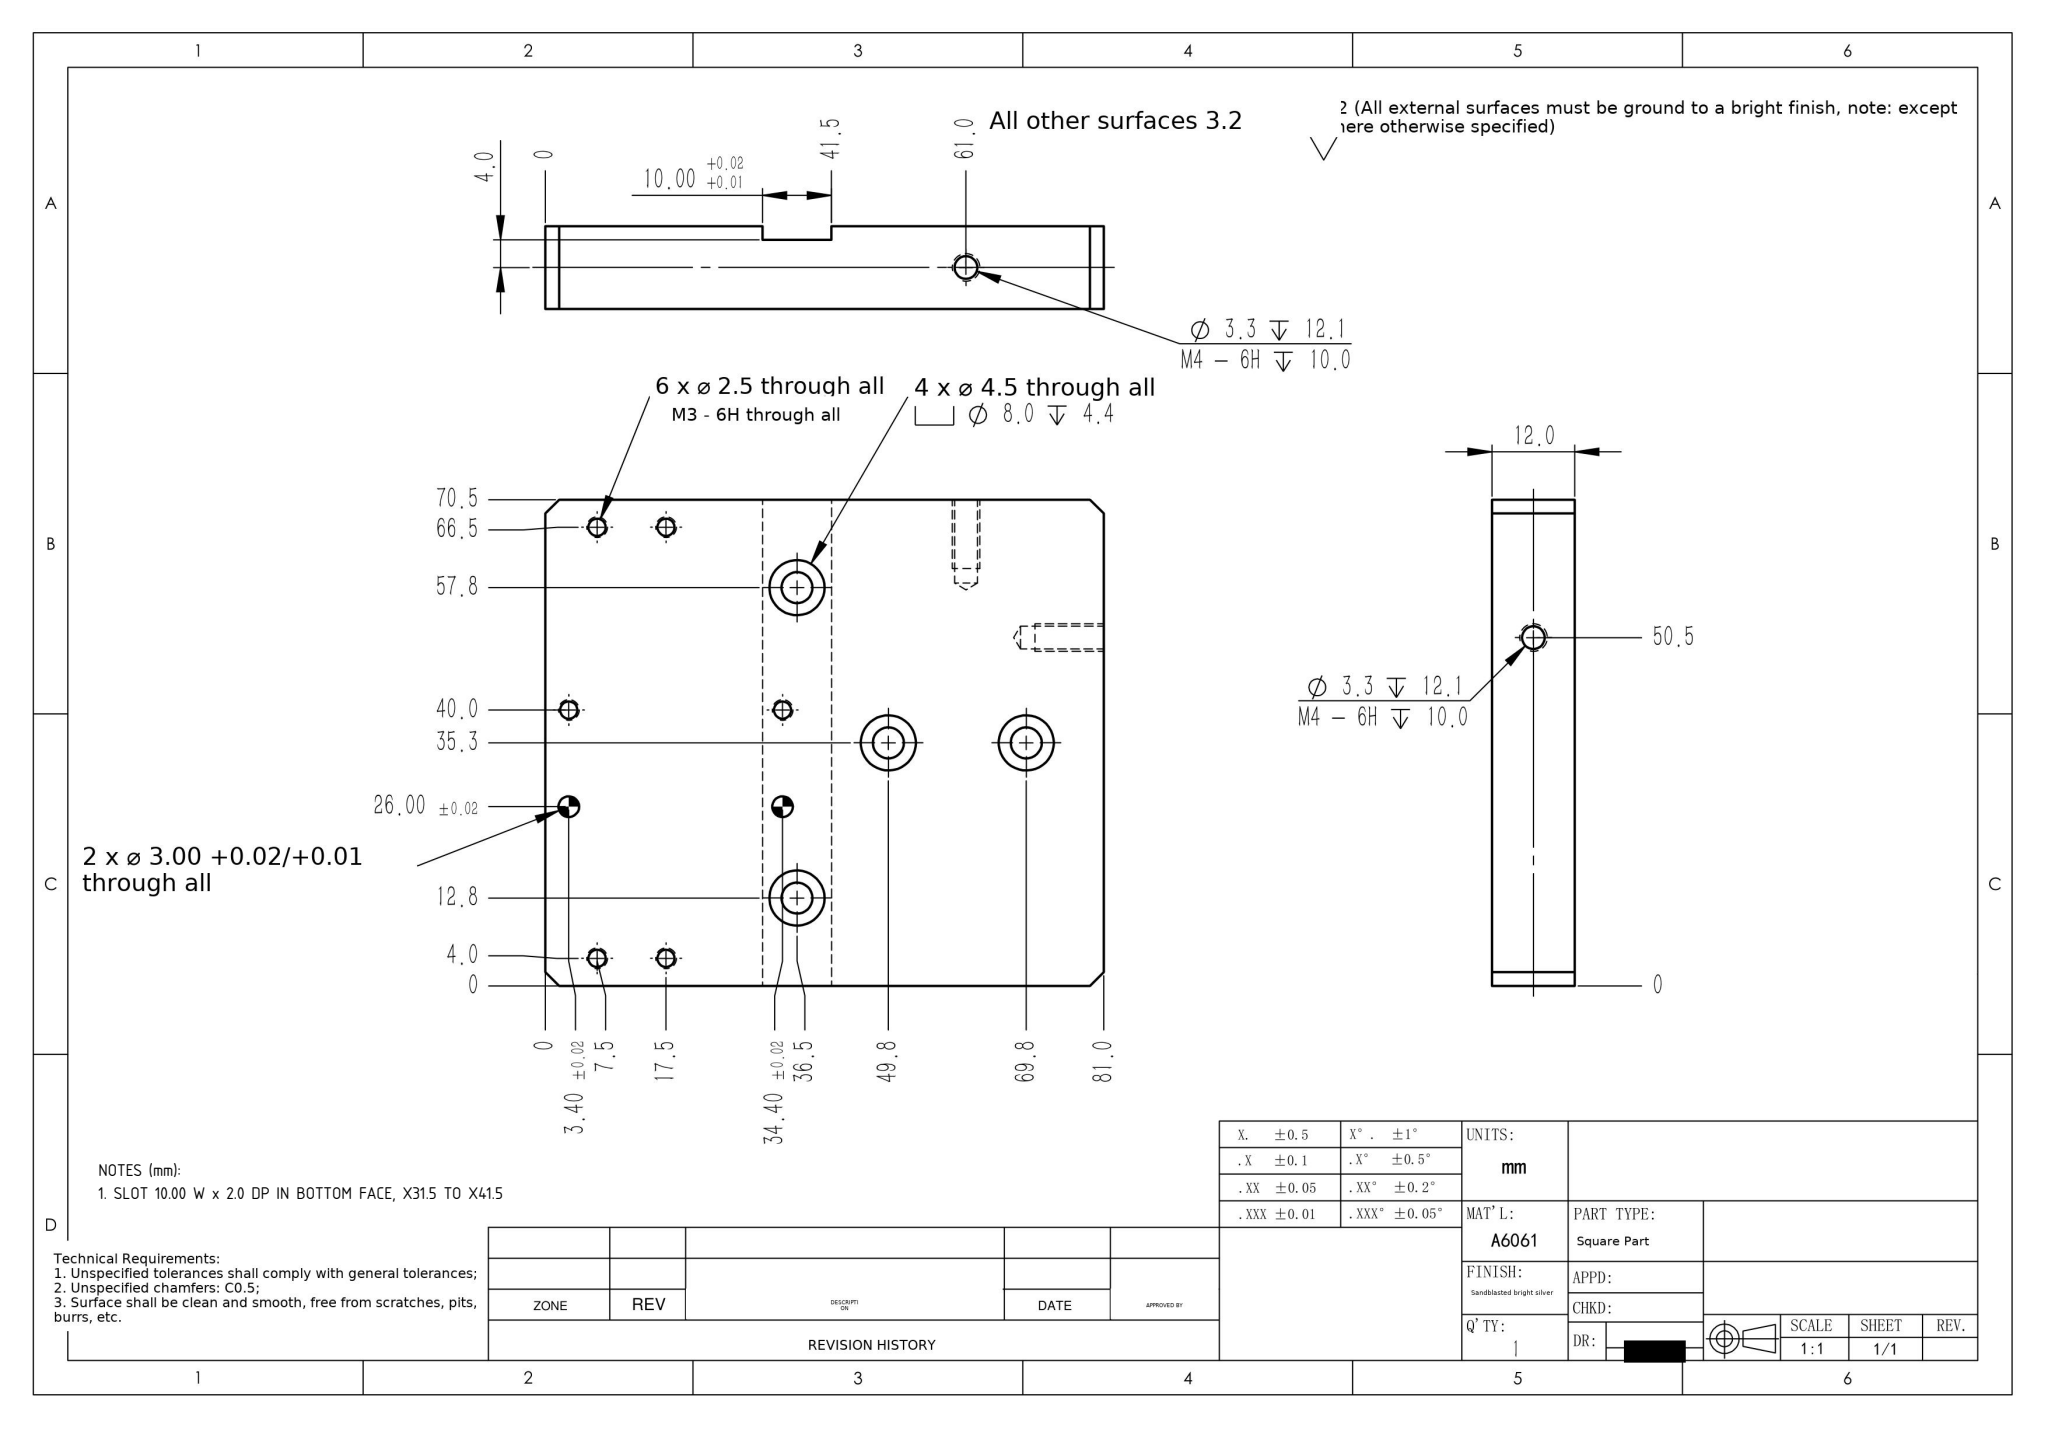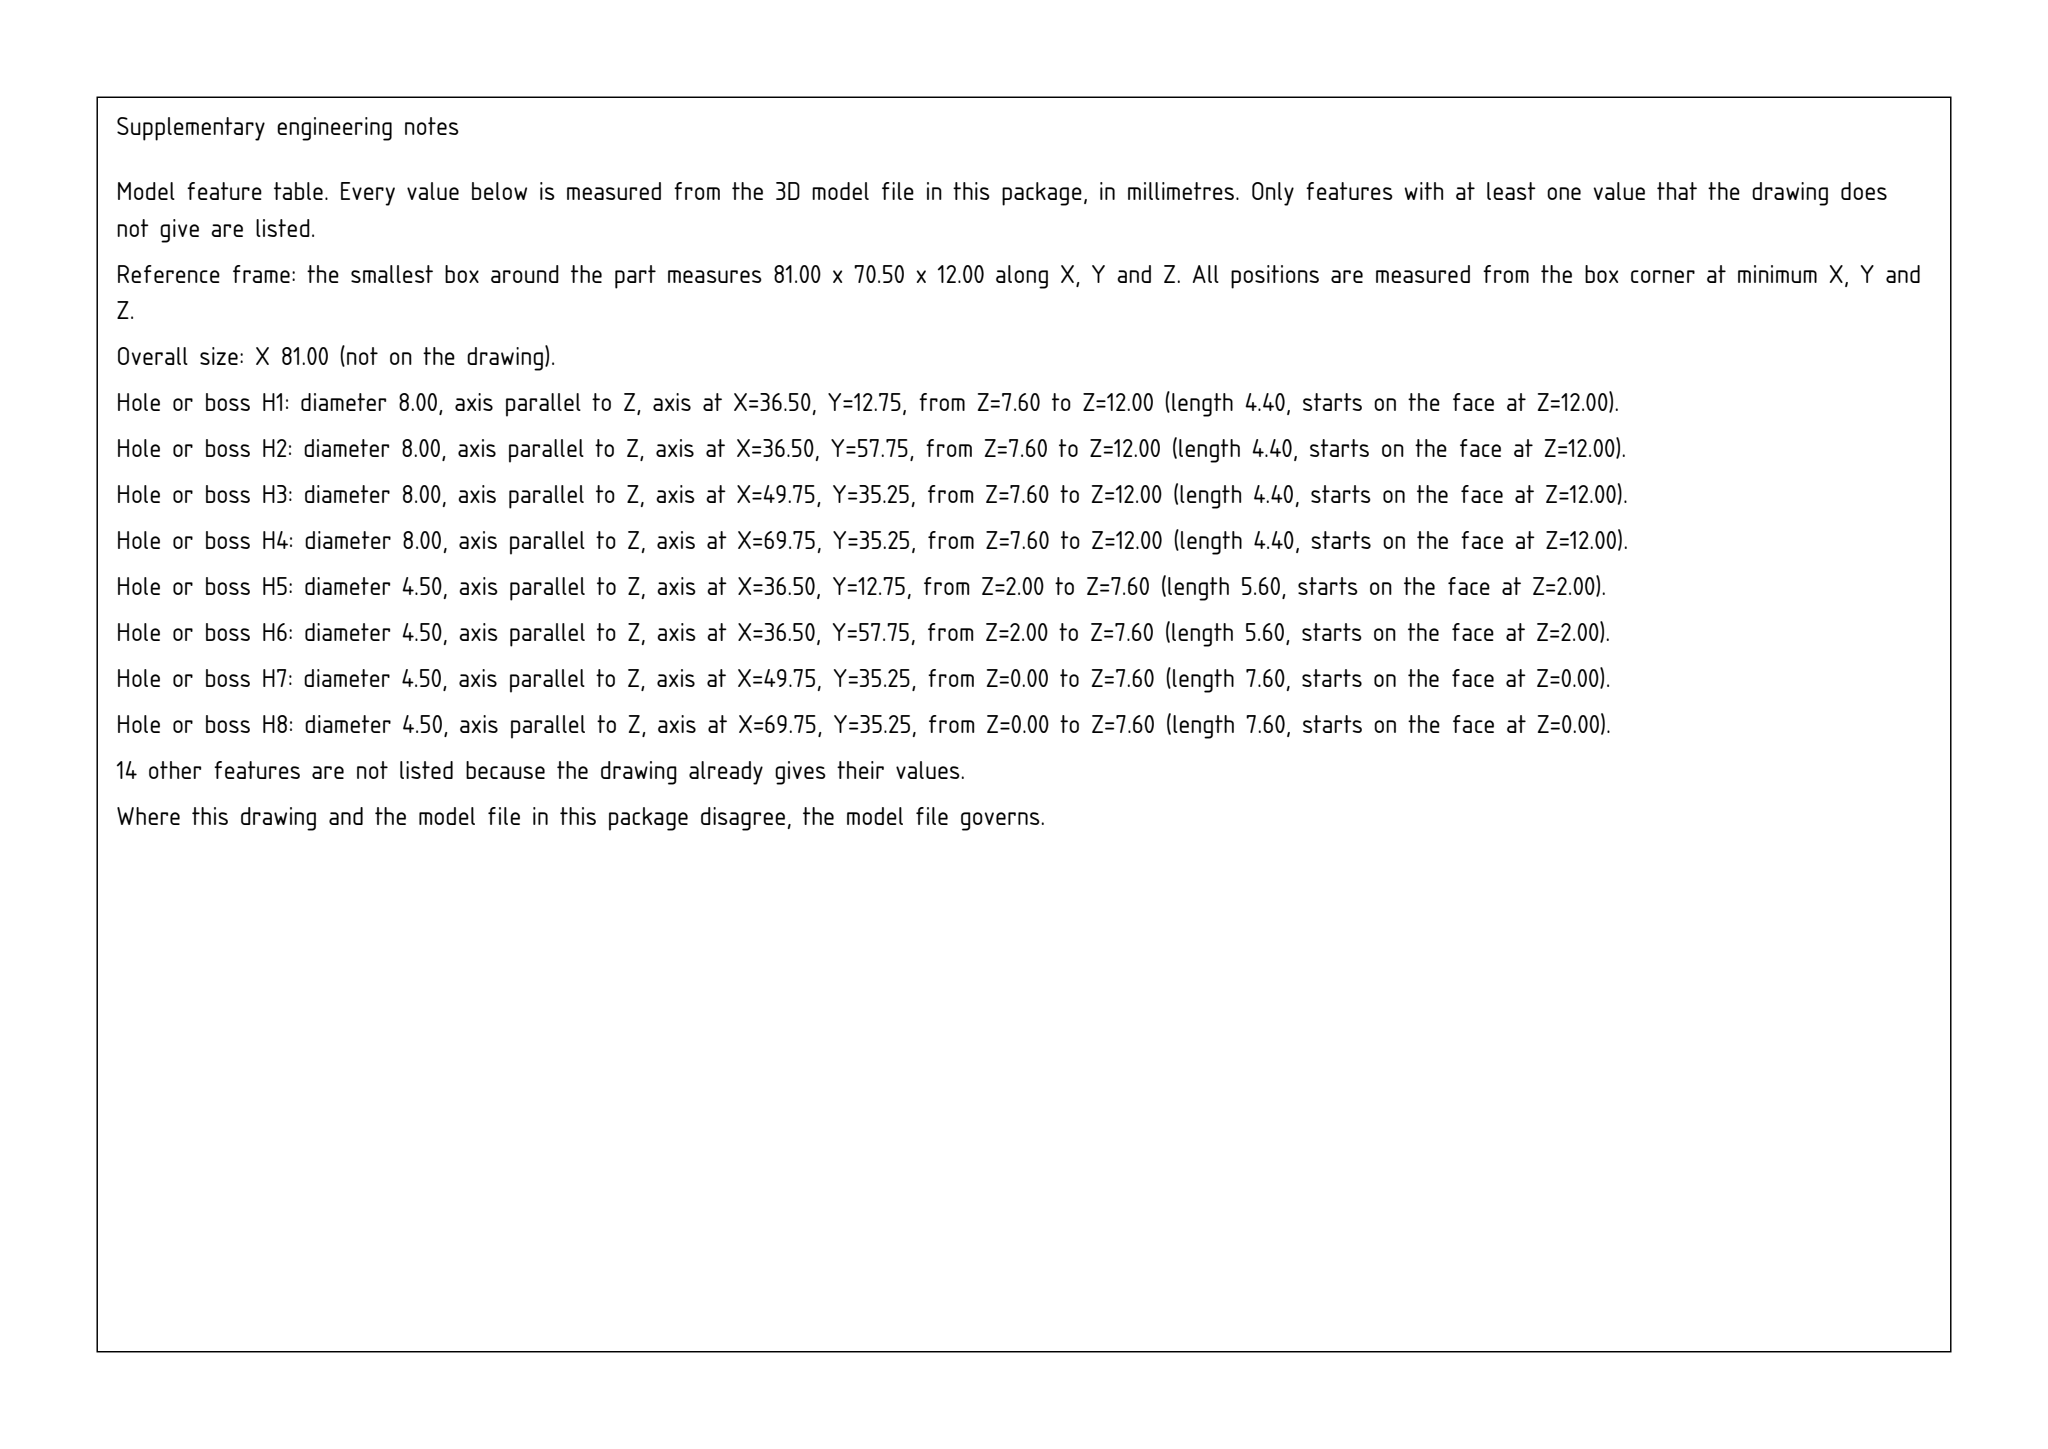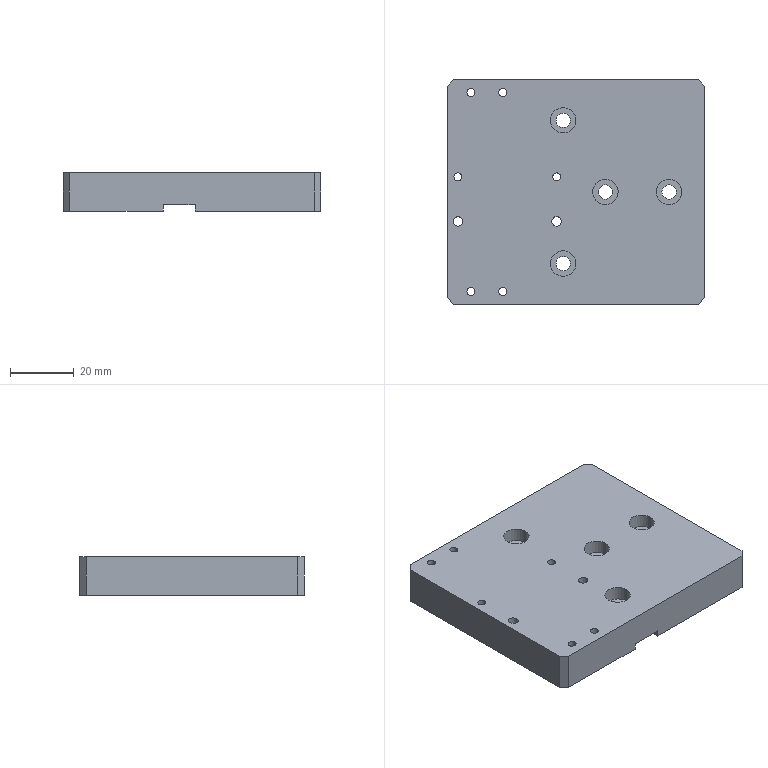Part | SolidWorks | mm | 1 solid | 58 faces | box 81 x 70.5 x 12 mm | volume 65004 mm3 | cylinder 36 | plane 18 | cone 4 | commonest cylinder face diameters 2.5 x12 8 x8 4.5 x8 3.3 x4 3 x4
Drawing notes:
SLOT 10.00 W x 2.0 DP IN BOTTOM FACE, X31.5 TO X41.5 | from the solid: x-planes 31.5 & 41.5 (10.00 wide); z-plane at 2.0 vs 12.0 thk = 2.0 DP cut from z=0 face; Ø2.5 at x=34.4 only 10.0 long and Ø4.5 at x=36.5 5.6 long under 4.4 CBORE (4.4+5.6=10.0)
build123d program:
from build123d import *

# Parameters (mm, degrees)
SKETCH1_W                                       = 81
SKETCH1_H                                       = 70.5
BOSS_EXTRUDE1_DEPTH                             = 12
M4_HEX_SOCKET_HEAD_CAP_SCREW_CBORE1_D           = 4.5
M4_HEX_SOCKET_HEAD_CAP_SCREW_CBORE1_CBORE_D     = 8
M4_HEX_SOCKET_HEAD_CAP_SCREW_CBORE1_CBORE_DEPTH = 4.4
M3_TAPPED_HOLE1_D                               = 2.5
SIZE_MM_DOWEL_PIN_HOLE1_D                       = 3
M4_TAPPED_HOLE1_D                               = 3.3
M4_TAPPED_HOLE1_DEPTH                           = 12.1
M4_TAPPED_HOLE1_TIP                             = 0.9914
M4_TAPPED_HOLE2_D                               = 3.3
M4_TAPPED_HOLE2_DEPTH                           = 12.1
M4_TAPPED_HOLE2_TIP                             = 0.9914
CHAMFER1_SIZE                                   = 2
SKETCH12_W                                      = 10
SKETCH12_H                                      = 70.5
CUT_EXTRUDE1_DEPTH                              = 2


with BuildPart() as part:
    # Sketch1 → Boss-Extrude1 (new body)
    with BuildSketch(Plane.XY):
        Rectangle(SKETCH1_W, SKETCH1_H)
    extrude(amount=BOSS_EXTRUDE1_DEPTH)

    # M4 Hex Socket Head Cap Screw CBORE1 (through all)
    with Locations(Plane.XY.offset(12)):
        with Locations((29.25, 0), (9.25, 0), (-4, 22.5), (-4, -22.5)):
            CounterBoreHole(M4_HEX_SOCKET_HEAD_CAP_SCREW_CBORE1_D / 2, M4_HEX_SOCKET_HEAD_CAP_SCREW_CBORE1_CBORE_D / 2, M4_HEX_SOCKET_HEAD_CAP_SCREW_CBORE1_CBORE_DEPTH)

    # M3 Tapped Hole1 (through all)
    with Locations(Plane.XY.offset(12)):
        with Locations((-33, 31.25), (-23, 31.25), (-23, -31.25), (-33, -31.25), (-37.1, 4.75), (-6.1, 4.75), (-68.1, 4.75)):
            Hole(M3_TAPPED_HOLE1_D / 2)

    # Size mm Dowel Pin Hole1 (through all)
    with Locations(Plane.XY.offset(12)):
        with Locations((-37.1, -9.25), (-6.1, -9.25)):
            Hole(SIZE_MM_DOWEL_PIN_HOLE1_D / 2)

    # M4 Tapped Hole1
    with Locations(Plane(origin=(0, 35.25, 0), x_dir=(1, 0, 0), z_dir=(0, 1, 0))):
        with Locations((20.5, -6)):
            Hole(M4_TAPPED_HOLE1_D / 2, depth=M4_TAPPED_HOLE1_DEPTH)
            with Locations((0, 0, -(M4_TAPPED_HOLE1_DEPTH + M4_TAPPED_HOLE1_TIP / 2))):  # 118° drill point
                Cone(0, M4_TAPPED_HOLE1_D / 2, M4_TAPPED_HOLE1_TIP, mode=Mode.SUBTRACT)

    # M4 Tapped Hole2
    with Locations(Plane(origin=(40.5, 0, 0), x_dir=(0, 0, -1), z_dir=(1, 0, 0))):
        with Locations((-6, 15.25)):
            Hole(M4_TAPPED_HOLE2_D / 2, depth=M4_TAPPED_HOLE2_DEPTH)
            with Locations((0, 0, -(M4_TAPPED_HOLE2_DEPTH + M4_TAPPED_HOLE2_TIP / 2))):  # 118° drill point
                Cone(0, M4_TAPPED_HOLE2_D / 2, M4_TAPPED_HOLE2_TIP, mode=Mode.SUBTRACT)

    # Chamfer1
    chamfer1_edges = [part.edges().sort_by_distance(p)[0] for p in [
        (40.5, -35.25, 6),
        (-40.5, -35.25, 6),
        (-40.5, 35.25, 6),
        (40.5, 35.25, 6),
    ]]
    chamfer(chamfer1_edges, length=CHAMFER1_SIZE)

    # Sketch12 → Cut-Extrude1 (cut)
    with BuildSketch(Plane(origin=(0, 0, 0), x_dir=(-1, 0, 0), z_dir=(0, 0, -1))):
        with Locations((4, 0)):
            Rectangle(SKETCH12_W, SKETCH12_H)
    extrude(amount=-CUT_EXTRUDE1_DEPTH, mode=Mode.SUBTRACT)


solid = part.part